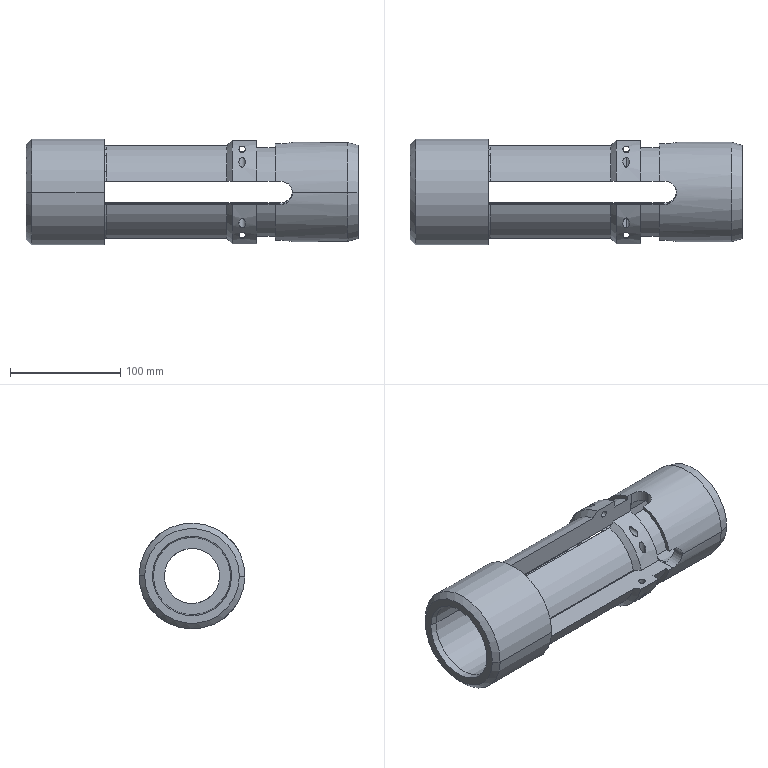Component | SolidWorks | 216InnerTubeAssembly-1_FishingBody-1 | 1 solid | 89 faces | volume 812152 mm3 | cylinder 50 | plane 25 | cone 10 | torus 4 | commonest cylinder face diameters 6 x16 21 x10 96 x6 70 x4 86 x4 83 x4 73.01 x2 90 x2 | material Alloy Steel